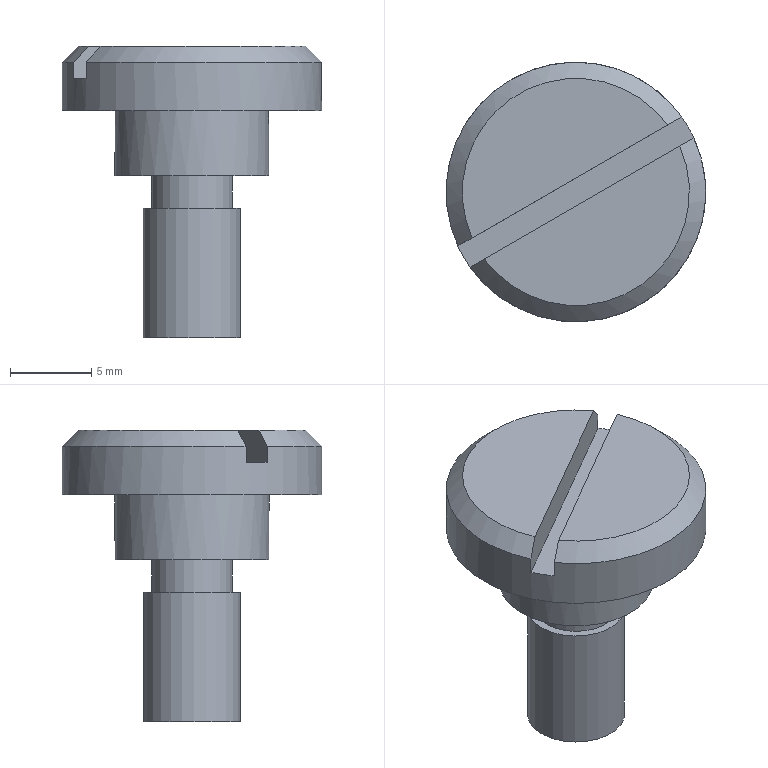Component | NX | DRILL_BUSH_SCREW | 1 solid | 15 faces | box 16 x 16 x 18 mm | volume 1283 mm3 | plane 9 | cylinder 4 | cone 2 | commonest cylinder face diameters 6 x1 5 x1 9.5 x1 16 x1
STEP:
#1=CARTESIAN_POINT('',(0.,0.,0.));
#2=DIRECTION('',(0.,0.,1.));
#3=DIRECTION('',(1.,0.,0.));
#4=AXIS2_PLACEMENT_3D('',#1,#2,#3);
#5=CARTESIAN_POINT('',(-27.652,33.976,178.));
#6=VERTEX_POINT('',#5);
#7=CARTESIAN_POINT('',(-15.598,40.935,178.));
#8=VERTEX_POINT('',#7);
#9=CARTESIAN_POINT('',(-31.151,31.956,178.));
#10=DIRECTION('',(0.866,0.5,0.));
#11=VECTOR('',#10,1.);
#12=LINE('',#9,#11);
#13=CARTESIAN_POINT('',(-22.,38.105,178.));
#14=DIRECTION('',(0.,0.,1.));
#15=DIRECTION('',(0.866,0.5,0.));
#16=AXIS2_PLACEMENT_3D('',#13,#14,#15);
#17=PLANE('',#16);
#18=CARTESIAN_POINT('',(-11.,-0.75));
#19=DIRECTION('',(1.,0.));
#20=VECTOR('',#19,1.);
#21=LINE('',#18,#20);
#22=(GEOMETRIC_REPRESENTATION_CONTEXT(2)PARAMETRIC_REPRESENTATION_CONTEXT()REPRESENTATION_CONTEXT('',''));
#23=DEFINITIONAL_REPRESENTATION('',(#21),#22);
#24=PCURVE('',#17,#23);
#25=CARTESIAN_POINT('',(-31.151,31.956,176.));
#26=DIRECTION('',(0.5,-0.866,0.));
#27=DIRECTION('',(0.,0.,-1.));
#28=AXIS2_PLACEMENT_3D('',#25,#26,#27);
#29=PLANE('',#28);
#30=CARTESIAN_POINT('',(-2.,0.));
#31=DIRECTION('',(0.,1.));
#32=VECTOR('',#31,1.);
#33=LINE('',#30,#32);
#34=(GEOMETRIC_REPRESENTATION_CONTEXT(2)PARAMETRIC_REPRESENTATION_CONTEXT()REPRESENTATION_CONTEXT('',''));
#35=DEFINITIONAL_REPRESENTATION('',(#33),#34);
#36=PCURVE('',#29,#35);
#37=SURFACE_CURVE('',#12,(#24,#36),.PCURVE_S1.);
#38=EDGE_CURVE('',#6,#8,#37,.T.);
#39=ORIENTED_EDGE('',*,*,#38,.F.);
#40=CARTESIAN_POINT('',(-22.,38.105,178.));
#41=DIRECTION('',(0.,0.,1.));
#42=DIRECTION('',(0.866,0.5,0.));
#43=AXIS2_PLACEMENT_3D('',#40,#41,#42);
#44=CIRCLE('',#43,7.);
#45=CARTESIAN_POINT('',(0.,0.));
#46=DIRECTION('',(1.,0.));
#47=AXIS2_PLACEMENT_2D('',#45,#46);
#48=CIRCLE('',#47,7.);
#49=(GEOMETRIC_REPRESENTATION_CONTEXT(2)PARAMETRIC_REPRESENTATION_CONTEXT()REPRESENTATION_CONTEXT('',''));
#50=DEFINITIONAL_REPRESENTATION('',(#48),#49);
#51=PCURVE('',#17,#50);
#52=CARTESIAN_POINT('',(-22.,38.105,177.));
#53=DIRECTION('',(0.,0.,-1.));
#54=DIRECTION('',(-0.866,-0.5,0.));
#55=AXIS2_PLACEMENT_3D('',#52,#53,#54);
#56=CONICAL_SURFACE('',#55,8.,0.7854);
#57=CARTESIAN_POINT('',(9.425,-1.));
#58=DIRECTION('',(-1.,0.));
#59=VECTOR('',#58,1.);
#60=LINE('',#57,#59);
#61=(GEOMETRIC_REPRESENTATION_CONTEXT(2)PARAMETRIC_REPRESENTATION_CONTEXT()REPRESENTATION_CONTEXT('',''));
#62=DEFINITIONAL_REPRESENTATION('',(#60),#61);
#63=PCURVE('',#56,#62);
#64=SURFACE_CURVE('',#44,(#51,#63),.PCURVE_S1.);
#65=EDGE_CURVE('',#6,#8,#64,.T.);
#66=ORIENTED_EDGE('',*,*,#65,.T.);
#67=EDGE_LOOP('',(#39,#66));
#68=FACE_BOUND('',#67,.T.);
#69=ADVANCED_FACE('',(#68),#17,.T.);
#70=CARTESIAN_POINT('',(-19.835,39.355,168.));
#71=VERTEX_POINT('',#70);
#72=CARTESIAN_POINT('',(-22.,38.105,168.));
#73=DIRECTION('',(0.,0.,1.));
#74=DIRECTION('',(0.866,0.5,0.));
#75=AXIS2_PLACEMENT_3D('',#72,#73,#74);
#76=CIRCLE('',#75,2.5);
#77=CARTESIAN_POINT('',(-22.,38.105,168.));
#78=DIRECTION('',(0.,0.,1.));
#79=DIRECTION('',(0.866,0.5,0.));
#80=AXIS2_PLACEMENT_3D('',#77,#78,#79);
#81=PLANE('',#80);
#82=CARTESIAN_POINT('',(0.,0.));
#83=DIRECTION('',(1.,-0.));
#84=AXIS2_PLACEMENT_2D('',#82,#83);
#85=CIRCLE('',#84,2.5);
#86=(GEOMETRIC_REPRESENTATION_CONTEXT(2)PARAMETRIC_REPRESENTATION_CONTEXT()REPRESENTATION_CONTEXT('',''));
#87=DEFINITIONAL_REPRESENTATION('',(#85),#86);
#88=PCURVE('',#81,#87);
#89=CARTESIAN_POINT('',(-22.,38.105,168.));
#90=DIRECTION('',(0.,0.,1.));
#91=DIRECTION('',(0.866,0.5,0.));
#92=AXIS2_PLACEMENT_3D('',#89,#90,#91);
#93=CYLINDRICAL_SURFACE('',#92,2.5);
#94=CARTESIAN_POINT('',(0.,0.));
#95=DIRECTION('',(1.,0.));
#96=VECTOR('',#95,1.);
#97=LINE('',#94,#96);
#98=(GEOMETRIC_REPRESENTATION_CONTEXT(2)PARAMETRIC_REPRESENTATION_CONTEXT()REPRESENTATION_CONTEXT('',''));
#99=DEFINITIONAL_REPRESENTATION('',(#97),#98);
#100=PCURVE('',#93,#99);
#101=SURFACE_CURVE('',#76,(#88,#100),.PCURVE_S1.);
#102=EDGE_CURVE('',#71,#71,#101,.T.);
#103=ORIENTED_EDGE('',*,*,#102,.F.);
#104=EDGE_LOOP('',(#103));
#105=FACE_BOUND('',#104,.T.);
#106=CARTESIAN_POINT('',(-19.402,39.605,168.));
#107=VERTEX_POINT('',#106);
#108=CARTESIAN_POINT('',(-22.,38.105,168.));
#109=DIRECTION('',(0.,0.,-1.));
#110=DIRECTION('',(0.866,0.5,0.));
#111=AXIS2_PLACEMENT_3D('',#108,#109,#110);
#112=CIRCLE('',#111,3.);
#113=CARTESIAN_POINT('',(3.,0.));
#114=CARTESIAN_POINT('',(3.,-5.196));
#115=CARTESIAN_POINT('',(-1.5,-2.598));
#116=CARTESIAN_POINT('',(-6.,-0.));
#117=CARTESIAN_POINT('',(-1.5,2.598));
#118=CARTESIAN_POINT('',(3.,5.196));
#119=CARTESIAN_POINT('',(3.,0.));
#120=(BOUNDED_CURVE()B_SPLINE_CURVE(2,(#113,#114,#115,#116,#117,#118,#119),.UNSPECIFIED.,.T.,.F.)B_SPLINE_CURVE_WITH_KNOTS((1,2,2,2,2,1),(-2.094,0.,2.094,4.189,6.283,8.378),.UNSPECIFIED.)CURVE()GEOMETRIC_REPRESENTATION_ITEM()RATIONAL_B_SPLINE_CURVE((1.,0.5,1.,0.5,1.,0.5,1.))REPRESENTATION_ITEM(''));
#121=(GEOMETRIC_REPRESENTATION_CONTEXT(2)PARAMETRIC_REPRESENTATION_CONTEXT()REPRESENTATION_CONTEXT('',''));
#122=DEFINITIONAL_REPRESENTATION('',(#120),#121);
#123=PCURVE('',#81,#122);
#124=CARTESIAN_POINT('',(-22.,38.105,160.));
#125=DIRECTION('',(0.,0.,1.));
#126=DIRECTION('',(0.866,0.5,0.));
#127=AXIS2_PLACEMENT_3D('',#124,#125,#126);
#128=CYLINDRICAL_SURFACE('',#127,3.);
#129=CARTESIAN_POINT('',(6.283,8.));
#130=DIRECTION('',(-1.,0.));
#131=VECTOR('',#130,1.);
#132=LINE('',#129,#131);
#133=(GEOMETRIC_REPRESENTATION_CONTEXT(2)PARAMETRIC_REPRESENTATION_CONTEXT()REPRESENTATION_CONTEXT('',''));
#134=DEFINITIONAL_REPRESENTATION('',(#132),#133);
#135=PCURVE('',#128,#134);
#136=SURFACE_CURVE('',#112,(#123,#135),.PCURVE_S1.);
#137=EDGE_CURVE('',#107,#107,#136,.T.);
#138=ORIENTED_EDGE('',*,*,#137,.F.);
#139=EDGE_LOOP('',(#138));
#140=FACE_BOUND('',#139,.T.);
#141=ADVANCED_FACE('',(#105,#140),#81,.T.);
#142=CARTESIAN_POINT('',(-19.402,39.605,160.));
#143=VERTEX_POINT('',#142);
#144=CARTESIAN_POINT('',(-22.,38.105,160.));
#145=DIRECTION('',(0.,0.,1.));
#146=DIRECTION('',(0.866,0.5,0.));
#147=AXIS2_PLACEMENT_3D('',#144,#145,#146);
#148=CIRCLE('',#147,3.);
#149=CARTESIAN_POINT('',(-22.,38.105,160.));
#150=DIRECTION('',(0.,0.,-1.));
#151=DIRECTION('',(-0.866,-0.5,0.));
#152=AXIS2_PLACEMENT_3D('',#149,#150,#151);
#153=PLANE('',#152);
#154=CARTESIAN_POINT('',(-3.,0.));
#155=CARTESIAN_POINT('',(-3.,5.196));
#156=CARTESIAN_POINT('',(1.5,2.598));
#157=CARTESIAN_POINT('',(6.,-0.));
#158=CARTESIAN_POINT('',(1.5,-2.598));
#159=CARTESIAN_POINT('',(-3.,-5.196));
#160=CARTESIAN_POINT('',(-3.,0.));
#161=(BOUNDED_CURVE()B_SPLINE_CURVE(2,(#154,#155,#156,#157,#158,#159,#160),.UNSPECIFIED.,.T.,.F.)B_SPLINE_CURVE_WITH_KNOTS((1,2,2,2,2,1),(-2.094,0.,2.094,4.189,6.283,8.378),.UNSPECIFIED.)CURVE()GEOMETRIC_REPRESENTATION_ITEM()RATIONAL_B_SPLINE_CURVE((1.,0.5,1.,0.5,1.,0.5,1.))REPRESENTATION_ITEM(''));
#162=(GEOMETRIC_REPRESENTATION_CONTEXT(2)PARAMETRIC_REPRESENTATION_CONTEXT()REPRESENTATION_CONTEXT('',''));
#163=DEFINITIONAL_REPRESENTATION('',(#161),#162);
#164=PCURVE('',#153,#163);
#165=CARTESIAN_POINT('',(0.,0.));
#166=DIRECTION('',(1.,0.));
#167=VECTOR('',#166,1.);
#168=LINE('',#165,#167);
#169=(GEOMETRIC_REPRESENTATION_CONTEXT(2)PARAMETRIC_REPRESENTATION_CONTEXT()REPRESENTATION_CONTEXT('',''));
#170=DEFINITIONAL_REPRESENTATION('',(#168),#169);
#171=PCURVE('',#128,#170);
#172=SURFACE_CURVE('',#148,(#164,#171),.PCURVE_S1.);
#173=EDGE_CURVE('',#143,#143,#172,.T.);
#174=ORIENTED_EDGE('',*,*,#173,.F.);
#175=EDGE_LOOP('',(#174));
#176=FACE_BOUND('',#175,.T.);
#177=ADVANCED_FACE('',(#176),#153,.T.);
#178=ORIENTED_EDGE('',*,*,#137,.T.);
#179=CARTESIAN_POINT('',(-19.402,39.605,160.));
#180=CARTESIAN_POINT('',(-19.402,39.605,168.));
#181=B_SPLINE_CURVE_WITH_KNOTS('',1,(#179,#180),.UNSPECIFIED.,.F.,.F.,(2,2),(0.,8.),.PIECEWISE_BEZIER_KNOTS.);
#182=CARTESIAN_POINT('',(0.,0.));
#183=DIRECTION('',(0.,1.));
#184=VECTOR('',#183,1.);
#185=LINE('',#182,#184);
#186=(GEOMETRIC_REPRESENTATION_CONTEXT(2)PARAMETRIC_REPRESENTATION_CONTEXT()REPRESENTATION_CONTEXT('',''));
#187=DEFINITIONAL_REPRESENTATION('',(#185),#186);
#188=PCURVE('',#128,#187);
#189=CARTESIAN_POINT('',(6.283,0.));
#190=DIRECTION('',(0.,1.));
#191=VECTOR('',#190,1.);
#192=LINE('',#189,#191);
#193=(GEOMETRIC_REPRESENTATION_CONTEXT(2)PARAMETRIC_REPRESENTATION_CONTEXT()REPRESENTATION_CONTEXT('',''));
#194=DEFINITIONAL_REPRESENTATION('',(#192),#193);
#195=PCURVE('',#128,#194);
#196=SEAM_CURVE('',#181,(#188,#195),.PCURVE_S1.);
#197=EDGE_CURVE('',#143,#107,#196,.T.);
#198=ORIENTED_EDGE('',*,*,#197,.F.);
#199=ORIENTED_EDGE('',*,*,#173,.T.);
#200=ORIENTED_EDGE('',*,*,#197,.T.);
#201=EDGE_LOOP('',(#178,#198,#199,#200));
#202=FACE_BOUND('',#201,.T.);
#203=ADVANCED_FACE('',(#202),#128,.T.);
#204=CARTESIAN_POINT('',(-19.835,39.355,170.));
#205=VERTEX_POINT('',#204);
#206=CARTESIAN_POINT('',(-24.165,36.855,170.));
#207=VERTEX_POINT('',#206);
#208=CARTESIAN_POINT('',(-22.,38.105,170.));
#209=DIRECTION('',(0.,0.,1.));
#210=DIRECTION('',(-0.866,-0.5,0.));
#211=AXIS2_PLACEMENT_3D('',#208,#209,#210);
#212=CIRCLE('',#211,2.5);
#213=CARTESIAN_POINT('',(-3.142,2.));
#214=DIRECTION('',(1.,0.));
#215=VECTOR('',#214,1.);
#216=LINE('',#213,#215);
#217=(GEOMETRIC_REPRESENTATION_CONTEXT(2)PARAMETRIC_REPRESENTATION_CONTEXT()REPRESENTATION_CONTEXT('',''));
#218=DEFINITIONAL_REPRESENTATION('',(#216),#217);
#219=PCURVE('',#93,#218);
#220=CARTESIAN_POINT('',(-22.,38.105,170.));
#221=DIRECTION('',(0.,0.,-1.));
#222=DIRECTION('',(-0.866,-0.5,0.));
#223=AXIS2_PLACEMENT_3D('',#220,#221,#222);
#224=PLANE('',#223);
#225=CARTESIAN_POINT('',(2.5,0.));
#226=CARTESIAN_POINT('',(2.5,-4.33));
#227=CARTESIAN_POINT('',(-1.25,-2.165));
#228=CARTESIAN_POINT('',(-5.,-0.));
#229=CARTESIAN_POINT('',(-1.25,2.165));
#230=CARTESIAN_POINT('',(2.5,4.33));
#231=CARTESIAN_POINT('',(2.5,0.));
#232=(BOUNDED_CURVE()B_SPLINE_CURVE(2,(#225,#226,#227,#228,#229,#230,#231),.UNSPECIFIED.,.T.,.F.)B_SPLINE_CURVE_WITH_KNOTS((1,2,2,2,2,1),(-2.094,0.,2.094,4.189,6.283,8.378),.UNSPECIFIED.)CURVE()GEOMETRIC_REPRESENTATION_ITEM()RATIONAL_B_SPLINE_CURVE((1.,0.5,1.,0.5,1.,0.5,1.))REPRESENTATION_ITEM(''));
#233=(GEOMETRIC_REPRESENTATION_CONTEXT(2)PARAMETRIC_REPRESENTATION_CONTEXT()REPRESENTATION_CONTEXT('',''));
#234=DEFINITIONAL_REPRESENTATION('',(#232),#233);
#235=PCURVE('',#224,#234);
#236=SURFACE_CURVE('',#212,(#219,#235),.PCURVE_S1.);
#237=EDGE_CURVE('',#205,#207,#236,.T.);
#238=ORIENTED_EDGE('',*,*,#237,.F.);
#239=CARTESIAN_POINT('',(-19.835,39.355,168.));
#240=CARTESIAN_POINT('',(-19.835,39.355,170.));
#241=B_SPLINE_CURVE_WITH_KNOTS('',1,(#239,#240),.UNSPECIFIED.,.F.,.F.,(2,2),(0.,2.),.PIECEWISE_BEZIER_KNOTS.);
#242=CARTESIAN_POINT('',(0.,0.));
#243=DIRECTION('',(0.,1.));
#244=VECTOR('',#243,1.);
#245=LINE('',#242,#244);
#246=(GEOMETRIC_REPRESENTATION_CONTEXT(2)PARAMETRIC_REPRESENTATION_CONTEXT()REPRESENTATION_CONTEXT('',''));
#247=DEFINITIONAL_REPRESENTATION('',(#245),#246);
#248=PCURVE('',#93,#247);
#249=CARTESIAN_POINT('',(6.283,0.));
#250=DIRECTION('',(0.,1.));
#251=VECTOR('',#250,1.);
#252=LINE('',#249,#251);
#253=(GEOMETRIC_REPRESENTATION_CONTEXT(2)PARAMETRIC_REPRESENTATION_CONTEXT()REPRESENTATION_CONTEXT('',''));
#254=DEFINITIONAL_REPRESENTATION('',(#252),#253);
#255=PCURVE('',#93,#254);
#256=SEAM_CURVE('',#241,(#248,#255),.PCURVE_S1.);
#257=EDGE_CURVE('',#71,#205,#256,.T.);
#258=ORIENTED_EDGE('',*,*,#257,.F.);
#259=ORIENTED_EDGE('',*,*,#102,.T.);
#260=ORIENTED_EDGE('',*,*,#257,.T.);
#261=CARTESIAN_POINT('',(-22.,38.105,170.));
#262=DIRECTION('',(0.,0.,1.));
#263=DIRECTION('',(-0.866,-0.5,0.));
#264=AXIS2_PLACEMENT_3D('',#261,#262,#263);
#265=CIRCLE('',#264,2.5);
#266=CARTESIAN_POINT('',(3.142,2.));
#267=DIRECTION('',(1.,0.));
#268=VECTOR('',#267,1.);
#269=LINE('',#266,#268);
#270=(GEOMETRIC_REPRESENTATION_CONTEXT(2)PARAMETRIC_REPRESENTATION_CONTEXT()REPRESENTATION_CONTEXT('',''));
#271=DEFINITIONAL_REPRESENTATION('',(#269),#270);
#272=PCURVE('',#93,#271);
#273=CARTESIAN_POINT('',(2.5,0.));
#274=CARTESIAN_POINT('',(2.5,-4.33));
#275=CARTESIAN_POINT('',(-1.25,-2.165));
#276=CARTESIAN_POINT('',(-5.,-0.));
#277=CARTESIAN_POINT('',(-1.25,2.165));
#278=CARTESIAN_POINT('',(2.5,4.33));
#279=CARTESIAN_POINT('',(2.5,0.));
#280=(BOUNDED_CURVE()B_SPLINE_CURVE(2,(#273,#274,#275,#276,#277,#278,#279),.UNSPECIFIED.,.T.,.F.)B_SPLINE_CURVE_WITH_KNOTS((1,2,2,2,2,1),(-2.094,0.,2.094,4.189,6.283,8.378),.UNSPECIFIED.)CURVE()GEOMETRIC_REPRESENTATION_ITEM()RATIONAL_B_SPLINE_CURVE((1.,0.5,1.,0.5,1.,0.5,1.))REPRESENTATION_ITEM(''));
#281=(GEOMETRIC_REPRESENTATION_CONTEXT(2)PARAMETRIC_REPRESENTATION_CONTEXT()REPRESENTATION_CONTEXT('',''));
#282=DEFINITIONAL_REPRESENTATION('',(#280),#281);
#283=PCURVE('',#224,#282);
#284=SURFACE_CURVE('',#265,(#272,#283),.PCURVE_S1.);
#285=EDGE_CURVE('',#207,#205,#284,.T.);
#286=ORIENTED_EDGE('',*,*,#285,.F.);
#287=EDGE_LOOP('',(#238,#258,#259,#260,#286));
#288=FACE_BOUND('',#287,.T.);
#289=ADVANCED_FACE('',(#288),#93,.T.);
#290=ORIENTED_EDGE('',*,*,#285,.T.);
#291=ORIENTED_EDGE('',*,*,#237,.T.);
#292=EDGE_LOOP('',(#290,#291));
#293=FACE_BOUND('',#292,.T.);
#294=CARTESIAN_POINT('',(-17.886,40.48,170.));
#295=VERTEX_POINT('',#294);
#296=CARTESIAN_POINT('',(-22.,38.105,170.));
#297=DIRECTION('',(0.,0.,1.));
#298=DIRECTION('',(0.866,0.5,0.));
#299=AXIS2_PLACEMENT_3D('',#296,#297,#298);
#300=CIRCLE('',#299,4.75);
#301=CARTESIAN_POINT('',(-4.75,0.));
#302=CARTESIAN_POINT('',(-4.75,8.227));
#303=CARTESIAN_POINT('',(2.375,4.114));
#304=CARTESIAN_POINT('',(9.5,0.));
#305=CARTESIAN_POINT('',(2.375,-4.114));
#306=CARTESIAN_POINT('',(-4.75,-8.227));
#307=CARTESIAN_POINT('',(-4.75,0.));
#308=(BOUNDED_CURVE()B_SPLINE_CURVE(2,(#301,#302,#303,#304,#305,#306,#307),.UNSPECIFIED.,.T.,.F.)B_SPLINE_CURVE_WITH_KNOTS((1,2,2,2,2,1),(-2.094,0.,2.094,4.189,6.283,8.378),.UNSPECIFIED.)CURVE()GEOMETRIC_REPRESENTATION_ITEM()RATIONAL_B_SPLINE_CURVE((1.,0.5,1.,0.5,1.,0.5,1.))REPRESENTATION_ITEM(''));
#309=(GEOMETRIC_REPRESENTATION_CONTEXT(2)PARAMETRIC_REPRESENTATION_CONTEXT()REPRESENTATION_CONTEXT('',''));
#310=DEFINITIONAL_REPRESENTATION('',(#308),#309);
#311=PCURVE('',#224,#310);
#312=CARTESIAN_POINT('',(-22.,38.105,170.));
#313=DIRECTION('',(0.,0.,1.));
#314=DIRECTION('',(0.866,0.5,0.));
#315=AXIS2_PLACEMENT_3D('',#312,#313,#314);
#316=CYLINDRICAL_SURFACE('',#315,4.75);
#317=CARTESIAN_POINT('',(0.,0.));
#318=DIRECTION('',(1.,0.));
#319=VECTOR('',#318,1.);
#320=LINE('',#317,#319);
#321=(GEOMETRIC_REPRESENTATION_CONTEXT(2)PARAMETRIC_REPRESENTATION_CONTEXT()REPRESENTATION_CONTEXT('',''));
#322=DEFINITIONAL_REPRESENTATION('',(#320),#321);
#323=PCURVE('',#316,#322);
#324=SURFACE_CURVE('',#300,(#311,#323),.PCURVE_S1.);
#325=EDGE_CURVE('',#295,#295,#324,.T.);
#326=ORIENTED_EDGE('',*,*,#325,.F.);
#327=EDGE_LOOP('',(#326));
#328=FACE_BOUND('',#327,.T.);
#329=ADVANCED_FACE('',(#293,#328),#224,.T.);
#330=CARTESIAN_POINT('',(-17.886,40.48,174.));
#331=VERTEX_POINT('',#330);
#332=CARTESIAN_POINT('',(-26.114,35.73,174.));
#333=VERTEX_POINT('',#332);
#334=CARTESIAN_POINT('',(-22.,38.105,174.));
#335=DIRECTION('',(0.,0.,1.));
#336=DIRECTION('',(-0.866,-0.5,0.));
#337=AXIS2_PLACEMENT_3D('',#334,#335,#336);
#338=CIRCLE('',#337,4.75);
#339=CARTESIAN_POINT('',(-3.142,4.));
#340=DIRECTION('',(1.,0.));
#341=VECTOR('',#340,1.);
#342=LINE('',#339,#341);
#343=(GEOMETRIC_REPRESENTATION_CONTEXT(2)PARAMETRIC_REPRESENTATION_CONTEXT()REPRESENTATION_CONTEXT('',''));
#344=DEFINITIONAL_REPRESENTATION('',(#342),#343);
#345=PCURVE('',#316,#344);
#346=CARTESIAN_POINT('',(-22.,38.105,174.));
#347=DIRECTION('',(0.,0.,-1.));
#348=DIRECTION('',(-0.866,-0.5,0.));
#349=AXIS2_PLACEMENT_3D('',#346,#347,#348);
#350=PLANE('',#349);
#351=CARTESIAN_POINT('',(4.75,0.));
#352=CARTESIAN_POINT('',(4.75,-8.227));
#353=CARTESIAN_POINT('',(-2.375,-4.114));
#354=CARTESIAN_POINT('',(-9.5,-0.));
#355=CARTESIAN_POINT('',(-2.375,4.114));
#356=CARTESIAN_POINT('',(4.75,8.227));
#357=CARTESIAN_POINT('',(4.75,0.));
#358=(BOUNDED_CURVE()B_SPLINE_CURVE(2,(#351,#352,#353,#354,#355,#356,#357),.UNSPECIFIED.,.T.,.F.)B_SPLINE_CURVE_WITH_KNOTS((1,2,2,2,2,1),(-2.094,0.,2.094,4.189,6.283,8.378),.UNSPECIFIED.)CURVE()GEOMETRIC_REPRESENTATION_ITEM()RATIONAL_B_SPLINE_CURVE((1.,0.5,1.,0.5,1.,0.5,1.))REPRESENTATION_ITEM(''));
#359=(GEOMETRIC_REPRESENTATION_CONTEXT(2)PARAMETRIC_REPRESENTATION_CONTEXT()REPRESENTATION_CONTEXT('',''));
#360=DEFINITIONAL_REPRESENTATION('',(#358),#359);
#361=PCURVE('',#350,#360);
#362=SURFACE_CURVE('',#338,(#345,#361),.PCURVE_S1.);
#363=EDGE_CURVE('',#331,#333,#362,.T.);
#364=ORIENTED_EDGE('',*,*,#363,.F.);
#365=CARTESIAN_POINT('',(-17.886,40.48,170.));
#366=CARTESIAN_POINT('',(-17.886,40.48,174.));
#367=B_SPLINE_CURVE_WITH_KNOTS('',1,(#365,#366),.UNSPECIFIED.,.F.,.F.,(2,2),(0.,4.),.PIECEWISE_BEZIER_KNOTS.);
#368=CARTESIAN_POINT('',(0.,0.));
#369=DIRECTION('',(0.,1.));
#370=VECTOR('',#369,1.);
#371=LINE('',#368,#370);
#372=(GEOMETRIC_REPRESENTATION_CONTEXT(2)PARAMETRIC_REPRESENTATION_CONTEXT()REPRESENTATION_CONTEXT('',''));
#373=DEFINITIONAL_REPRESENTATION('',(#371),#372);
#374=PCURVE('',#316,#373);
#375=CARTESIAN_POINT('',(6.283,0.));
#376=DIRECTION('',(0.,1.));
#377=VECTOR('',#376,1.);
#378=LINE('',#375,#377);
#379=(GEOMETRIC_REPRESENTATION_CONTEXT(2)PARAMETRIC_REPRESENTATION_CONTEXT()REPRESENTATION_CONTEXT('',''));
#380=DEFINITIONAL_REPRESENTATION('',(#378),#379);
#381=PCURVE('',#316,#380);
#382=SEAM_CURVE('',#367,(#374,#381),.PCURVE_S1.);
#383=EDGE_CURVE('',#295,#331,#382,.T.);
#384=ORIENTED_EDGE('',*,*,#383,.F.);
#385=ORIENTED_EDGE('',*,*,#325,.T.);
#386=ORIENTED_EDGE('',*,*,#383,.T.);
#387=CARTESIAN_POINT('',(-22.,38.105,174.));
#388=DIRECTION('',(0.,0.,1.));
#389=DIRECTION('',(-0.866,-0.5,0.));
#390=AXIS2_PLACEMENT_3D('',#387,#388,#389);
#391=CIRCLE('',#390,4.75);
#392=CARTESIAN_POINT('',(3.142,4.));
#393=DIRECTION('',(1.,0.));
#394=VECTOR('',#393,1.);
#395=LINE('',#392,#394);
#396=(GEOMETRIC_REPRESENTATION_CONTEXT(2)PARAMETRIC_REPRESENTATION_CONTEXT()REPRESENTATION_CONTEXT('',''));
#397=DEFINITIONAL_REPRESENTATION('',(#395),#396);
#398=PCURVE('',#316,#397);
#399=CARTESIAN_POINT('',(4.75,0.));
#400=CARTESIAN_POINT('',(4.75,-8.227));
#401=CARTESIAN_POINT('',(-2.375,-4.114));
#402=CARTESIAN_POINT('',(-9.5,-0.));
#403=CARTESIAN_POINT('',(-2.375,4.114));
#404=CARTESIAN_POINT('',(4.75,8.227));
#405=CARTESIAN_POINT('',(4.75,0.));
#406=(BOUNDED_CURVE()B_SPLINE_CURVE(2,(#399,#400,#401,#402,#403,#404,#405),.UNSPECIFIED.,.T.,.F.)B_SPLINE_CURVE_WITH_KNOTS((1,2,2,2,2,1),(-2.094,0.,2.094,4.189,6.283,8.378),.UNSPECIFIED.)CURVE()GEOMETRIC_REPRESENTATION_ITEM()RATIONAL_B_SPLINE_CURVE((1.,0.5,1.,0.5,1.,0.5,1.))REPRESENTATION_ITEM(''));
#407=(GEOMETRIC_REPRESENTATION_CONTEXT(2)PARAMETRIC_REPRESENTATION_CONTEXT()REPRESENTATION_CONTEXT('',''));
#408=DEFINITIONAL_REPRESENTATION('',(#406),#407);
#409=PCURVE('',#350,#408);
#410=SURFACE_CURVE('',#391,(#398,#409),.PCURVE_S1.);
#411=EDGE_CURVE('',#333,#331,#410,.T.);
#412=ORIENTED_EDGE('',*,*,#411,.F.);
#413=EDGE_LOOP('',(#364,#384,#385,#386,#412));
#414=FACE_BOUND('',#413,.T.);
#415=ADVANCED_FACE('',(#414),#316,.T.);
#416=CARTESIAN_POINT('',(-16.348,42.234,178.));
#417=VERTEX_POINT('',#416);
#418=CARTESIAN_POINT('',(-28.402,35.275,178.));
#419=VERTEX_POINT('',#418);
#420=CARTESIAN_POINT('',(-12.849,44.255,178.));
#421=DIRECTION('',(-0.866,-0.5,0.));
#422=VECTOR('',#421,1.);
#423=LINE('',#420,#422);
#424=CARTESIAN_POINT('',(-22.,38.105,178.));
#425=DIRECTION('',(0.,0.,1.));
#426=DIRECTION('',(0.866,0.5,0.));
#427=AXIS2_PLACEMENT_3D('',#424,#425,#426);
#428=PLANE('',#427);
#429=CARTESIAN_POINT('',(11.,0.75));
#430=DIRECTION('',(-1.,0.));
#431=VECTOR('',#430,1.);
#432=LINE('',#429,#431);
#433=(GEOMETRIC_REPRESENTATION_CONTEXT(2)PARAMETRIC_REPRESENTATION_CONTEXT()REPRESENTATION_CONTEXT('',''));
#434=DEFINITIONAL_REPRESENTATION('',(#432),#433);
#435=PCURVE('',#428,#434);
#436=CARTESIAN_POINT('',(-12.849,44.255,176.));
#437=DIRECTION('',(-0.5,0.866,0.));
#438=DIRECTION('',(0.,0.,1.));
#439=AXIS2_PLACEMENT_3D('',#436,#437,#438);
#440=PLANE('',#439);
#441=CARTESIAN_POINT('',(2.,0.));
#442=DIRECTION('',(0.,-1.));
#443=VECTOR('',#442,1.);
#444=LINE('',#441,#443);
#445=(GEOMETRIC_REPRESENTATION_CONTEXT(2)PARAMETRIC_REPRESENTATION_CONTEXT()REPRESENTATION_CONTEXT('',''));
#446=DEFINITIONAL_REPRESENTATION('',(#444),#445);
#447=PCURVE('',#440,#446);
#448=SURFACE_CURVE('',#423,(#435,#447),.PCURVE_S1.);
#449=EDGE_CURVE('',#417,#419,#448,.T.);
#450=ORIENTED_EDGE('',*,*,#449,.F.);
#451=CARTESIAN_POINT('',(-22.,38.105,178.));
#452=DIRECTION('',(0.,0.,1.));
#453=DIRECTION('',(0.866,0.5,0.));
#454=AXIS2_PLACEMENT_3D('',#451,#452,#453);
#455=CIRCLE('',#454,7.);
#456=CARTESIAN_POINT('',(0.,0.));
#457=DIRECTION('',(1.,0.));
#458=AXIS2_PLACEMENT_2D('',#456,#457);
#459=CIRCLE('',#458,7.);
#460=(GEOMETRIC_REPRESENTATION_CONTEXT(2)PARAMETRIC_REPRESENTATION_CONTEXT()REPRESENTATION_CONTEXT('',''));
#461=DEFINITIONAL_REPRESENTATION('',(#459),#460);
#462=PCURVE('',#428,#461);
#463=CARTESIAN_POINT('',(-22.,38.105,177.));
#464=DIRECTION('',(0.,0.,-1.));
#465=DIRECTION('',(-0.866,-0.5,0.));
#466=AXIS2_PLACEMENT_3D('',#463,#464,#465);
#467=CONICAL_SURFACE('',#466,8.,0.7854);
#468=CARTESIAN_POINT('',(3.142,-1.));
#469=DIRECTION('',(-1.,0.));
#470=VECTOR('',#469,1.);
#471=LINE('',#468,#470);
#472=(GEOMETRIC_REPRESENTATION_CONTEXT(2)PARAMETRIC_REPRESENTATION_CONTEXT()REPRESENTATION_CONTEXT('',''));
#473=DEFINITIONAL_REPRESENTATION('',(#471),#472);
#474=PCURVE('',#467,#473);
#475=SURFACE_CURVE('',#455,(#462,#474),.PCURVE_S1.);
#476=EDGE_CURVE('',#417,#419,#475,.T.);
#477=ORIENTED_EDGE('',*,*,#476,.T.);
#478=EDGE_LOOP('',(#450,#477));
#479=FACE_BOUND('',#478,.T.);
#480=ADVANCED_FACE('',(#479),#428,.T.);
#481=ORIENTED_EDGE('',*,*,#411,.T.);
#482=ORIENTED_EDGE('',*,*,#363,.T.);
#483=EDGE_LOOP('',(#481,#482));
#484=FACE_BOUND('',#483,.T.);
#485=CARTESIAN_POINT('',(-15.072,42.105,174.));
#486=VERTEX_POINT('',#485);
#487=CARTESIAN_POINT('',(-22.,38.105,174.));
#488=DIRECTION('',(0.,0.,1.));
#489=DIRECTION('',(0.866,0.5,0.));
#490=AXIS2_PLACEMENT_3D('',#487,#488,#489);
#491=CIRCLE('',#490,8.);
#492=CARTESIAN_POINT('',(-8.,0.));
#493=CARTESIAN_POINT('',(-8.,13.856));
#494=CARTESIAN_POINT('',(4.,6.928));
#495=CARTESIAN_POINT('',(16.,0.));
#496=CARTESIAN_POINT('',(4.,-6.928));
#497=CARTESIAN_POINT('',(-8.,-13.856));
#498=CARTESIAN_POINT('',(-8.,0.));
#499=(BOUNDED_CURVE()B_SPLINE_CURVE(2,(#492,#493,#494,#495,#496,#497,#498),.UNSPECIFIED.,.T.,.F.)B_SPLINE_CURVE_WITH_KNOTS((1,2,2,2,2,1),(-2.094,0.,2.094,4.189,6.283,8.378),.UNSPECIFIED.)CURVE()GEOMETRIC_REPRESENTATION_ITEM()RATIONAL_B_SPLINE_CURVE((1.,0.5,1.,0.5,1.,0.5,1.))REPRESENTATION_ITEM(''));
#500=(GEOMETRIC_REPRESENTATION_CONTEXT(2)PARAMETRIC_REPRESENTATION_CONTEXT()REPRESENTATION_CONTEXT('',''));
#501=DEFINITIONAL_REPRESENTATION('',(#499),#500);
#502=PCURVE('',#350,#501);
#503=CARTESIAN_POINT('',(-22.,38.105,174.));
#504=DIRECTION('',(0.,0.,1.));
#505=DIRECTION('',(0.866,0.5,0.));
#506=AXIS2_PLACEMENT_3D('',#503,#504,#505);
#507=CYLINDRICAL_SURFACE('',#506,8.);
#508=CARTESIAN_POINT('',(0.,0.));
#509=DIRECTION('',(1.,0.));
#510=VECTOR('',#509,1.);
#511=LINE('',#508,#510);
#512=(GEOMETRIC_REPRESENTATION_CONTEXT(2)PARAMETRIC_REPRESENTATION_CONTEXT()REPRESENTATION_CONTEXT('',''));
#513=DEFINITIONAL_REPRESENTATION('',(#511),#512);
#514=PCURVE('',#507,#513);
#515=SURFACE_CURVE('',#491,(#502,#514),.PCURVE_S1.);
#516=EDGE_CURVE('',#486,#486,#515,.T.);
#517=ORIENTED_EDGE('',*,*,#516,.F.);
#518=EDGE_LOOP('',(#517));
#519=FACE_BOUND('',#518,.T.);
#520=ADVANCED_FACE('',(#484,#519),#350,.T.);
#521=CARTESIAN_POINT('',(-14.727,41.438,177.));
#522=VERTEX_POINT('',#521);
#523=CARTESIAN_POINT('',(-14.727,41.438,176.));
#524=VERTEX_POINT('',#523);
#525=CARTESIAN_POINT('',(-14.727,41.438,174.));
#526=DIRECTION('',(0.,0.,-1.));
#527=VECTOR('',#526,1.);
#528=LINE('',#525,#527);
#529=CARTESIAN_POINT('',(6.189,0.));
#530=DIRECTION('',(0.,-1.));
#531=VECTOR('',#530,1.);
#532=LINE('',#529,#531);
#533=(GEOMETRIC_REPRESENTATION_CONTEXT(2)PARAMETRIC_REPRESENTATION_CONTEXT()REPRESENTATION_CONTEXT('',''));
#534=DEFINITIONAL_REPRESENTATION('',(#532),#533);
#535=PCURVE('',#507,#534);
#536=CARTESIAN_POINT('',(2.,18.965));
#537=DIRECTION('',(1.,0.));
#538=VECTOR('',#537,1.);
#539=LINE('',#536,#538);
#540=(GEOMETRIC_REPRESENTATION_CONTEXT(2)PARAMETRIC_REPRESENTATION_CONTEXT()REPRESENTATION_CONTEXT('',''));
#541=DEFINITIONAL_REPRESENTATION('',(#539),#540);
#542=PCURVE('',#29,#541);
#543=SURFACE_CURVE('',#528,(#535,#542),.PCURVE_S1.);
#544=EDGE_CURVE('',#522,#524,#543,.T.);
#545=ORIENTED_EDGE('',*,*,#544,.F.);
#546=CARTESIAN_POINT('',(-28.523,33.473,177.));
#547=VERTEX_POINT('',#546);
#548=CARTESIAN_POINT('',(-22.,38.105,177.));
#549=DIRECTION('',(0.,0.,-1.));
#550=DIRECTION('',(0.866,0.5,0.));
#551=AXIS2_PLACEMENT_3D('',#548,#549,#550);
#552=CIRCLE('',#551,8.);
#553=CARTESIAN_POINT('',(6.283,3.));
#554=DIRECTION('',(-1.,0.));
#555=VECTOR('',#554,1.);
#556=LINE('',#553,#555);
#557=(GEOMETRIC_REPRESENTATION_CONTEXT(2)PARAMETRIC_REPRESENTATION_CONTEXT()REPRESENTATION_CONTEXT('',''));
#558=DEFINITIONAL_REPRESENTATION('',(#556),#557);
#559=PCURVE('',#507,#558);
#560=CARTESIAN_POINT('',(3.142,0.));
#561=DIRECTION('',(1.,-0.));
#562=VECTOR('',#561,1.);
#563=LINE('',#560,#562);
#564=(GEOMETRIC_REPRESENTATION_CONTEXT(2)PARAMETRIC_REPRESENTATION_CONTEXT()REPRESENTATION_CONTEXT('',''));
#565=DEFINITIONAL_REPRESENTATION('',(#563),#564);
#566=PCURVE('',#56,#565);
#567=SURFACE_CURVE('',#552,(#559,#566),.PCURVE_S1.);
#568=EDGE_CURVE('',#522,#547,#567,.T.);
#569=ORIENTED_EDGE('',*,*,#568,.T.);
#570=CARTESIAN_POINT('',(-28.523,33.473,176.));
#571=VERTEX_POINT('',#570);
#572=CARTESIAN_POINT('',(-28.523,33.473,174.));
#573=DIRECTION('',(0.,0.,1.));
#574=VECTOR('',#573,1.);
#575=LINE('',#572,#574);
#576=CARTESIAN_POINT('',(3.235,0.));
#577=DIRECTION('',(0.,1.));
#578=VECTOR('',#577,1.);
#579=LINE('',#576,#578);
#580=(GEOMETRIC_REPRESENTATION_CONTEXT(2)PARAMETRIC_REPRESENTATION_CONTEXT()REPRESENTATION_CONTEXT('',''));
#581=DEFINITIONAL_REPRESENTATION('',(#579),#580);
#582=PCURVE('',#507,#581);
#583=CARTESIAN_POINT('',(2.,3.035));
#584=DIRECTION('',(-1.,0.));
#585=VECTOR('',#584,1.);
#586=LINE('',#583,#585);
#587=(GEOMETRIC_REPRESENTATION_CONTEXT(2)PARAMETRIC_REPRESENTATION_CONTEXT()REPRESENTATION_CONTEXT('',''));
#588=DEFINITIONAL_REPRESENTATION('',(#586),#587);
#589=PCURVE('',#29,#588);
#590=SURFACE_CURVE('',#575,(#582,#589),.PCURVE_S1.);
#591=EDGE_CURVE('',#571,#547,#590,.T.);
#592=ORIENTED_EDGE('',*,*,#591,.F.);
#593=CARTESIAN_POINT('',(-29.273,34.772,176.));
#594=VERTEX_POINT('',#593);
#595=CARTESIAN_POINT('',(-22.,38.105,176.));
#596=DIRECTION('',(0.,0.,-1.));
#597=DIRECTION('',(0.866,0.5,0.));
#598=AXIS2_PLACEMENT_3D('',#595,#596,#597);
#599=CIRCLE('',#598,8.);
#600=CARTESIAN_POINT('',(6.283,2.));
#601=DIRECTION('',(-1.,0.));
#602=VECTOR('',#601,1.);
#603=LINE('',#600,#602);
#604=(GEOMETRIC_REPRESENTATION_CONTEXT(2)PARAMETRIC_REPRESENTATION_CONTEXT()REPRESENTATION_CONTEXT('',''));
#605=DEFINITIONAL_REPRESENTATION('',(#603),#604);
#606=PCURVE('',#507,#605);
#607=CARTESIAN_POINT('',(-22.,38.105,176.));
#608=DIRECTION('',(0.,0.,1.));
#609=DIRECTION('',(0.866,0.5,0.));
#610=AXIS2_PLACEMENT_3D('',#607,#608,#609);
#611=PLANE('',#610);
#612=CARTESIAN_POINT('',(8.,0.));
#613=CARTESIAN_POINT('',(8.,-13.856));
#614=CARTESIAN_POINT('',(-4.,-6.928));
#615=CARTESIAN_POINT('',(-16.,-0.));
#616=CARTESIAN_POINT('',(-4.,6.928));
#617=CARTESIAN_POINT('',(8.,13.856));
#618=CARTESIAN_POINT('',(8.,0.));
#619=(BOUNDED_CURVE()B_SPLINE_CURVE(2,(#612,#613,#614,#615,#616,#617,#618),.UNSPECIFIED.,.T.,.F.)B_SPLINE_CURVE_WITH_KNOTS((1,2,2,2,2,1),(-2.094,0.,2.094,4.189,6.283,8.378),.UNSPECIFIED.)CURVE()GEOMETRIC_REPRESENTATION_ITEM()RATIONAL_B_SPLINE_CURVE((1.,0.5,1.,0.5,1.,0.5,1.))REPRESENTATION_ITEM(''));
#620=(GEOMETRIC_REPRESENTATION_CONTEXT(2)PARAMETRIC_REPRESENTATION_CONTEXT()REPRESENTATION_CONTEXT('',''));
#621=DEFINITIONAL_REPRESENTATION('',(#619),#620);
#622=PCURVE('',#611,#621);
#623=SURFACE_CURVE('',#599,(#606,#622),.PCURVE_S1.);
#624=EDGE_CURVE('',#571,#594,#623,.T.);
#625=ORIENTED_EDGE('',*,*,#624,.T.);
#626=CARTESIAN_POINT('',(-29.273,34.772,177.));
#627=VERTEX_POINT('',#626);
#628=CARTESIAN_POINT('',(-29.273,34.772,174.));
#629=DIRECTION('',(0.,0.,-1.));
#630=VECTOR('',#629,1.);
#631=LINE('',#628,#630);
#632=CARTESIAN_POINT('',(3.048,0.));
#633=DIRECTION('',(0.,-1.));
#634=VECTOR('',#633,1.);
#635=LINE('',#632,#634);
#636=(GEOMETRIC_REPRESENTATION_CONTEXT(2)PARAMETRIC_REPRESENTATION_CONTEXT()REPRESENTATION_CONTEXT('',''));
#637=DEFINITIONAL_REPRESENTATION('',(#635),#636);
#638=PCURVE('',#507,#637);
#639=CARTESIAN_POINT('',(-2.,-18.965));
#640=DIRECTION('',(-1.,0.));
#641=VECTOR('',#640,1.);
#642=LINE('',#639,#641);
#643=(GEOMETRIC_REPRESENTATION_CONTEXT(2)PARAMETRIC_REPRESENTATION_CONTEXT()REPRESENTATION_CONTEXT('',''));
#644=DEFINITIONAL_REPRESENTATION('',(#642),#643);
#645=PCURVE('',#440,#644);
#646=SURFACE_CURVE('',#631,(#638,#645),.PCURVE_S1.);
#647=EDGE_CURVE('',#627,#594,#646,.T.);
#648=ORIENTED_EDGE('',*,*,#647,.F.);
#649=CARTESIAN_POINT('',(-15.477,42.737,177.));
#650=VERTEX_POINT('',#649);
#651=CARTESIAN_POINT('',(-22.,38.105,177.));
#652=DIRECTION('',(0.,0.,-1.));
#653=DIRECTION('',(0.866,0.5,0.));
#654=AXIS2_PLACEMENT_3D('',#651,#652,#653);
#655=CIRCLE('',#654,8.);
#656=CARTESIAN_POINT('',(6.283,3.));
#657=DIRECTION('',(-1.,0.));
#658=VECTOR('',#657,1.);
#659=LINE('',#656,#658);
#660=(GEOMETRIC_REPRESENTATION_CONTEXT(2)PARAMETRIC_REPRESENTATION_CONTEXT()REPRESENTATION_CONTEXT('',''));
#661=DEFINITIONAL_REPRESENTATION('',(#659),#660);
#662=PCURVE('',#507,#661);
#663=CARTESIAN_POINT('',(-3.142,-0.));
#664=DIRECTION('',(1.,0.));
#665=VECTOR('',#664,1.);
#666=LINE('',#663,#665);
#667=(GEOMETRIC_REPRESENTATION_CONTEXT(2)PARAMETRIC_REPRESENTATION_CONTEXT()REPRESENTATION_CONTEXT('',''));
#668=DEFINITIONAL_REPRESENTATION('',(#666),#667);
#669=PCURVE('',#467,#668);
#670=SURFACE_CURVE('',#655,(#662,#669),.PCURVE_S1.);
#671=EDGE_CURVE('',#627,#650,#670,.T.);
#672=ORIENTED_EDGE('',*,*,#671,.T.);
#673=CARTESIAN_POINT('',(-15.477,42.737,176.));
#674=VERTEX_POINT('',#673);
#675=CARTESIAN_POINT('',(-15.477,42.737,174.));
#676=DIRECTION('',(0.,0.,1.));
#677=VECTOR('',#676,1.);
#678=LINE('',#675,#677);
#679=CARTESIAN_POINT('',(0.09389,0.));
#680=DIRECTION('',(0.,1.));
#681=VECTOR('',#680,1.);
#682=LINE('',#679,#681);
#683=(GEOMETRIC_REPRESENTATION_CONTEXT(2)PARAMETRIC_REPRESENTATION_CONTEXT()REPRESENTATION_CONTEXT('',''));
#684=DEFINITIONAL_REPRESENTATION('',(#682),#683);
#685=PCURVE('',#507,#684);
#686=CARTESIAN_POINT('',(-2.,-3.035));
#687=DIRECTION('',(1.,0.));
#688=VECTOR('',#687,1.);
#689=LINE('',#686,#688);
#690=(GEOMETRIC_REPRESENTATION_CONTEXT(2)PARAMETRIC_REPRESENTATION_CONTEXT()REPRESENTATION_CONTEXT('',''));
#691=DEFINITIONAL_REPRESENTATION('',(#689),#690);
#692=PCURVE('',#440,#691);
#693=SURFACE_CURVE('',#678,(#685,#692),.PCURVE_S1.);
#694=EDGE_CURVE('',#674,#650,#693,.T.);
#695=ORIENTED_EDGE('',*,*,#694,.F.);
#696=CARTESIAN_POINT('',(-15.072,42.105,176.));
#697=VERTEX_POINT('',#696);
#698=CARTESIAN_POINT('',(-22.,38.105,176.));
#699=DIRECTION('',(0.,0.,-1.));
#700=DIRECTION('',(0.866,0.5,0.));
#701=AXIS2_PLACEMENT_3D('',#698,#699,#700);
#702=CIRCLE('',#701,8.);
#703=CARTESIAN_POINT('',(6.283,2.));
#704=DIRECTION('',(-1.,0.));
#705=VECTOR('',#704,1.);
#706=LINE('',#703,#705);
#707=(GEOMETRIC_REPRESENTATION_CONTEXT(2)PARAMETRIC_REPRESENTATION_CONTEXT()REPRESENTATION_CONTEXT('',''));
#708=DEFINITIONAL_REPRESENTATION('',(#706),#707);
#709=PCURVE('',#507,#708);
#710=CARTESIAN_POINT('',(8.,0.));
#711=CARTESIAN_POINT('',(8.,-13.856));
#712=CARTESIAN_POINT('',(-4.,-6.928));
#713=CARTESIAN_POINT('',(-16.,-0.));
#714=CARTESIAN_POINT('',(-4.,6.928));
#715=CARTESIAN_POINT('',(8.,13.856));
#716=CARTESIAN_POINT('',(8.,0.));
#717=(BOUNDED_CURVE()B_SPLINE_CURVE(2,(#710,#711,#712,#713,#714,#715,#716),.UNSPECIFIED.,.T.,.F.)B_SPLINE_CURVE_WITH_KNOTS((1,2,2,2,2,1),(-2.094,0.,2.094,4.189,6.283,8.378),.UNSPECIFIED.)CURVE()GEOMETRIC_REPRESENTATION_ITEM()RATIONAL_B_SPLINE_CURVE((1.,0.5,1.,0.5,1.,0.5,1.))REPRESENTATION_ITEM(''));
#718=(GEOMETRIC_REPRESENTATION_CONTEXT(2)PARAMETRIC_REPRESENTATION_CONTEXT()REPRESENTATION_CONTEXT('',''));
#719=DEFINITIONAL_REPRESENTATION('',(#717),#718);
#720=PCURVE('',#611,#719);
#721=SURFACE_CURVE('',#702,(#709,#720),.PCURVE_S1.);
#722=EDGE_CURVE('',#674,#697,#721,.T.);
#723=ORIENTED_EDGE('',*,*,#722,.T.);
#724=CARTESIAN_POINT('',(-15.072,42.105,174.));
#725=CARTESIAN_POINT('',(-15.072,42.105,176.));
#726=B_SPLINE_CURVE_WITH_KNOTS('',1,(#724,#725),.UNSPECIFIED.,.F.,.F.,(2,2),(0.,2.),.PIECEWISE_BEZIER_KNOTS.);
#727=CARTESIAN_POINT('',(0.,0.));
#728=DIRECTION('',(0.,1.));
#729=VECTOR('',#728,1.);
#730=LINE('',#727,#729);
#731=(GEOMETRIC_REPRESENTATION_CONTEXT(2)PARAMETRIC_REPRESENTATION_CONTEXT()REPRESENTATION_CONTEXT('',''));
#732=DEFINITIONAL_REPRESENTATION('',(#730),#731);
#733=PCURVE('',#507,#732);
#734=CARTESIAN_POINT('',(6.283,0.));
#735=DIRECTION('',(0.,1.));
#736=VECTOR('',#735,1.);
#737=LINE('',#734,#736);
#738=(GEOMETRIC_REPRESENTATION_CONTEXT(2)PARAMETRIC_REPRESENTATION_CONTEXT()REPRESENTATION_CONTEXT('',''));
#739=DEFINITIONAL_REPRESENTATION('',(#737),#738);
#740=PCURVE('',#507,#739);
#741=SEAM_CURVE('',#726,(#733,#740),.PCURVE_S1.);
#742=EDGE_CURVE('',#486,#697,#741,.T.);
#743=ORIENTED_EDGE('',*,*,#742,.F.);
#744=ORIENTED_EDGE('',*,*,#516,.T.);
#745=ORIENTED_EDGE('',*,*,#742,.T.);
#746=CARTESIAN_POINT('',(-22.,38.105,176.));
#747=DIRECTION('',(0.,0.,-1.));
#748=DIRECTION('',(0.866,0.5,0.));
#749=AXIS2_PLACEMENT_3D('',#746,#747,#748);
#750=CIRCLE('',#749,8.);
#751=CARTESIAN_POINT('',(12.566,2.));
#752=DIRECTION('',(-1.,0.));
#753=VECTOR('',#752,1.);
#754=LINE('',#751,#753);
#755=(GEOMETRIC_REPRESENTATION_CONTEXT(2)PARAMETRIC_REPRESENTATION_CONTEXT()REPRESENTATION_CONTEXT('',''));
#756=DEFINITIONAL_REPRESENTATION('',(#754),#755);
#757=PCURVE('',#507,#756);
#758=CARTESIAN_POINT('',(8.,0.));
#759=CARTESIAN_POINT('',(8.,-13.856));
#760=CARTESIAN_POINT('',(-4.,-6.928));
#761=CARTESIAN_POINT('',(-16.,-0.));
#762=CARTESIAN_POINT('',(-4.,6.928));
#763=CARTESIAN_POINT('',(8.,13.856));
#764=CARTESIAN_POINT('',(8.,0.));
#765=(BOUNDED_CURVE()B_SPLINE_CURVE(2,(#758,#759,#760,#761,#762,#763,#764),.UNSPECIFIED.,.T.,.F.)B_SPLINE_CURVE_WITH_KNOTS((1,2,2,2,2,1),(-2.094,0.,2.094,4.189,6.283,8.378),.UNSPECIFIED.)CURVE()GEOMETRIC_REPRESENTATION_ITEM()RATIONAL_B_SPLINE_CURVE((1.,0.5,1.,0.5,1.,0.5,1.))REPRESENTATION_ITEM(''));
#766=(GEOMETRIC_REPRESENTATION_CONTEXT(2)PARAMETRIC_REPRESENTATION_CONTEXT()REPRESENTATION_CONTEXT('',''));
#767=DEFINITIONAL_REPRESENTATION('',(#765),#766);
#768=PCURVE('',#611,#767);
#769=SURFACE_CURVE('',#750,(#757,#768),.PCURVE_S1.);
#770=EDGE_CURVE('',#697,#524,#769,.T.);
#771=ORIENTED_EDGE('',*,*,#770,.T.);
#772=EDGE_LOOP('',(#545,#569,#592,#625,#648,#672,#695,#723,#743,#744,#745,#771));
#773=FACE_BOUND('',#772,.T.);
#774=ADVANCED_FACE('',(#773),#507,.T.);
#775=ORIENTED_EDGE('',*,*,#591,.T.);
#776=CARTESIAN_POINT('',(-28.523,33.473,177.));
#777=CARTESIAN_POINT('',(-28.233,33.641,177.333));
#778=CARTESIAN_POINT('',(-27.943,33.808,177.667));
#779=CARTESIAN_POINT('',(-27.652,33.976,178.));
#780=B_SPLINE_CURVE_WITH_KNOTS('',3,(#776,#777,#778,#779),.UNSPECIFIED.,.F.,.F.,(4,4),(0.,1.),.PIECEWISE_BEZIER_KNOTS.);
#781=CARTESIAN_POINT('',(-1.,3.035));
#782=CARTESIAN_POINT('',(-1.333,3.37));
#783=CARTESIAN_POINT('',(-1.667,3.705));
#784=CARTESIAN_POINT('',(-2.,4.04));
#785=B_SPLINE_CURVE_WITH_KNOTS('',3,(#781,#782,#783,#784),.UNSPECIFIED.,.F.,.F.,(4,4),(0.,1.),.PIECEWISE_BEZIER_KNOTS.);
#786=(GEOMETRIC_REPRESENTATION_CONTEXT(2)PARAMETRIC_REPRESENTATION_CONTEXT()REPRESENTATION_CONTEXT('',''));
#787=DEFINITIONAL_REPRESENTATION('',(#785),#786);
#788=PCURVE('',#29,#787);
#789=CARTESIAN_POINT('',(6.189,-0.));
#790=CARTESIAN_POINT('',(6.176,-1.));
#791=B_SPLINE_CURVE_WITH_KNOTS('',1,(#789,#790),.UNSPECIFIED.,.F.,.F.,(2,2),(0.,1.),.PIECEWISE_BEZIER_KNOTS.);
#792=(GEOMETRIC_REPRESENTATION_CONTEXT(2)PARAMETRIC_REPRESENTATION_CONTEXT()REPRESENTATION_CONTEXT('',''));
#793=DEFINITIONAL_REPRESENTATION('',(#791),#792);
#794=PCURVE('',#56,#793);
#795=SURFACE_CURVE('',#780,(#788,#794),.PCURVE_S1.);
#796=EDGE_CURVE('',#547,#6,#795,.T.);
#797=ORIENTED_EDGE('',*,*,#796,.T.);
#798=ORIENTED_EDGE('',*,*,#38,.T.);
#799=CARTESIAN_POINT('',(-15.598,40.935,178.));
#800=CARTESIAN_POINT('',(-15.307,41.103,177.667));
#801=CARTESIAN_POINT('',(-15.017,41.271,177.333));
#802=CARTESIAN_POINT('',(-14.727,41.438,177.));
#803=B_SPLINE_CURVE_WITH_KNOTS('',3,(#799,#800,#801,#802),.UNSPECIFIED.,.F.,.F.,(4,4),(0.,1.),.PIECEWISE_BEZIER_KNOTS.);
#804=CARTESIAN_POINT('',(-2.,17.96));
#805=CARTESIAN_POINT('',(-1.667,18.295));
#806=CARTESIAN_POINT('',(-1.333,18.63));
#807=CARTESIAN_POINT('',(-1.,18.965));
#808=B_SPLINE_CURVE_WITH_KNOTS('',3,(#804,#805,#806,#807),.UNSPECIFIED.,.F.,.F.,(4,4),(0.,1.),.PIECEWISE_BEZIER_KNOTS.);
#809=(GEOMETRIC_REPRESENTATION_CONTEXT(2)PARAMETRIC_REPRESENTATION_CONTEXT()REPRESENTATION_CONTEXT('',''));
#810=DEFINITIONAL_REPRESENTATION('',(#808),#809);
#811=PCURVE('',#29,#810);
#812=CARTESIAN_POINT('',(3.249,-1.));
#813=CARTESIAN_POINT('',(3.235,0.));
#814=B_SPLINE_CURVE_WITH_KNOTS('',1,(#812,#813),.UNSPECIFIED.,.F.,.F.,(2,2),(0.,1.),.PIECEWISE_BEZIER_KNOTS.);
#815=(GEOMETRIC_REPRESENTATION_CONTEXT(2)PARAMETRIC_REPRESENTATION_CONTEXT()REPRESENTATION_CONTEXT('',''));
#816=DEFINITIONAL_REPRESENTATION('',(#814),#815);
#817=PCURVE('',#56,#816);
#818=SURFACE_CURVE('',#803,(#811,#817),.PCURVE_S1.);
#819=EDGE_CURVE('',#8,#522,#818,.T.);
#820=ORIENTED_EDGE('',*,*,#819,.T.);
#821=ORIENTED_EDGE('',*,*,#544,.T.);
#822=CARTESIAN_POINT('',(-31.151,31.956,176.));
#823=DIRECTION('',(-0.866,-0.5,0.));
#824=VECTOR('',#823,1.);
#825=LINE('',#822,#824);
#826=CARTESIAN_POINT('',(0.,0.));
#827=DIRECTION('',(0.,-1.));
#828=VECTOR('',#827,1.);
#829=LINE('',#826,#828);
#830=(GEOMETRIC_REPRESENTATION_CONTEXT(2)PARAMETRIC_REPRESENTATION_CONTEXT()REPRESENTATION_CONTEXT('',''));
#831=DEFINITIONAL_REPRESENTATION('',(#829),#830);
#832=PCURVE('',#29,#831);
#833=CARTESIAN_POINT('',(-11.,-0.75));
#834=DIRECTION('',(-1.,0.));
#835=VECTOR('',#834,1.);
#836=LINE('',#833,#835);
#837=(GEOMETRIC_REPRESENTATION_CONTEXT(2)PARAMETRIC_REPRESENTATION_CONTEXT()REPRESENTATION_CONTEXT('',''));
#838=DEFINITIONAL_REPRESENTATION('',(#836),#837);
#839=PCURVE('',#611,#838);
#840=SURFACE_CURVE('',#825,(#832,#839),.PCURVE_S1.);
#841=EDGE_CURVE('',#524,#571,#840,.T.);
#842=ORIENTED_EDGE('',*,*,#841,.T.);
#843=EDGE_LOOP('',(#775,#797,#798,#820,#821,#842));
#844=FACE_BOUND('',#843,.T.);
#845=ADVANCED_FACE('',(#844),#29,.F.);
#846=ORIENTED_EDGE('',*,*,#694,.T.);
#847=CARTESIAN_POINT('',(-15.477,42.737,177.));
#848=CARTESIAN_POINT('',(-15.767,42.57,177.333));
#849=CARTESIAN_POINT('',(-16.057,42.402,177.667));
#850=CARTESIAN_POINT('',(-16.348,42.234,178.));
#851=B_SPLINE_CURVE_WITH_KNOTS('',3,(#847,#848,#849,#850),.UNSPECIFIED.,.F.,.F.,(4,4),(0.,1.),.PIECEWISE_BEZIER_KNOTS.);
#852=CARTESIAN_POINT('',(1.,-3.035));
#853=CARTESIAN_POINT('',(1.333,-3.37));
#854=CARTESIAN_POINT('',(1.667,-3.705));
#855=CARTESIAN_POINT('',(2.,-4.04));
#856=B_SPLINE_CURVE_WITH_KNOTS('',3,(#852,#853,#854,#855),.UNSPECIFIED.,.F.,.F.,(4,4),(0.,1.),.PIECEWISE_BEZIER_KNOTS.);
#857=(GEOMETRIC_REPRESENTATION_CONTEXT(2)PARAMETRIC_REPRESENTATION_CONTEXT()REPRESENTATION_CONTEXT('',''));
#858=DEFINITIONAL_REPRESENTATION('',(#856),#857);
#859=PCURVE('',#440,#858);
#860=CARTESIAN_POINT('',(3.048,-0.));
#861=CARTESIAN_POINT('',(3.034,-1.));
#862=B_SPLINE_CURVE_WITH_KNOTS('',1,(#860,#861),.UNSPECIFIED.,.F.,.F.,(2,2),(0.,1.),.PIECEWISE_BEZIER_KNOTS.);
#863=(GEOMETRIC_REPRESENTATION_CONTEXT(2)PARAMETRIC_REPRESENTATION_CONTEXT()REPRESENTATION_CONTEXT('',''));
#864=DEFINITIONAL_REPRESENTATION('',(#862),#863);
#865=PCURVE('',#467,#864);
#866=SURFACE_CURVE('',#851,(#859,#865),.PCURVE_S1.);
#867=EDGE_CURVE('',#650,#417,#866,.T.);
#868=ORIENTED_EDGE('',*,*,#867,.T.);
#869=ORIENTED_EDGE('',*,*,#449,.T.);
#870=CARTESIAN_POINT('',(-28.402,35.275,178.));
#871=CARTESIAN_POINT('',(-28.693,35.107,177.667));
#872=CARTESIAN_POINT('',(-28.983,34.94,177.333));
#873=CARTESIAN_POINT('',(-29.273,34.772,177.));
#874=B_SPLINE_CURVE_WITH_KNOTS('',3,(#870,#871,#872,#873),.UNSPECIFIED.,.F.,.F.,(4,4),(0.,1.),.PIECEWISE_BEZIER_KNOTS.);
#875=CARTESIAN_POINT('',(2.,-17.96));
#876=CARTESIAN_POINT('',(1.667,-18.295));
#877=CARTESIAN_POINT('',(1.333,-18.63));
#878=CARTESIAN_POINT('',(1.,-18.965));
#879=B_SPLINE_CURVE_WITH_KNOTS('',3,(#875,#876,#877,#878),.UNSPECIFIED.,.F.,.F.,(4,4),(0.,1.),.PIECEWISE_BEZIER_KNOTS.);
#880=(GEOMETRIC_REPRESENTATION_CONTEXT(2)PARAMETRIC_REPRESENTATION_CONTEXT()REPRESENTATION_CONTEXT('',''));
#881=DEFINITIONAL_REPRESENTATION('',(#879),#880);
#882=PCURVE('',#440,#881);
#883=CARTESIAN_POINT('',(0.1073,-1.));
#884=CARTESIAN_POINT('',(0.09389,-0.));
#885=B_SPLINE_CURVE_WITH_KNOTS('',1,(#883,#884),.UNSPECIFIED.,.F.,.F.,(2,2),(0.,1.),.PIECEWISE_BEZIER_KNOTS.);
#886=(GEOMETRIC_REPRESENTATION_CONTEXT(2)PARAMETRIC_REPRESENTATION_CONTEXT()REPRESENTATION_CONTEXT('',''));
#887=DEFINITIONAL_REPRESENTATION('',(#885),#886);
#888=PCURVE('',#467,#887);
#889=SURFACE_CURVE('',#874,(#882,#888),.PCURVE_S1.);
#890=EDGE_CURVE('',#419,#627,#889,.T.);
#891=ORIENTED_EDGE('',*,*,#890,.T.);
#892=ORIENTED_EDGE('',*,*,#647,.T.);
#893=CARTESIAN_POINT('',(-12.849,44.255,176.));
#894=DIRECTION('',(0.866,0.5,0.));
#895=VECTOR('',#894,1.);
#896=LINE('',#893,#895);
#897=CARTESIAN_POINT('',(0.,0.));
#898=DIRECTION('',(0.,1.));
#899=VECTOR('',#898,1.);
#900=LINE('',#897,#899);
#901=(GEOMETRIC_REPRESENTATION_CONTEXT(2)PARAMETRIC_REPRESENTATION_CONTEXT()REPRESENTATION_CONTEXT('',''));
#902=DEFINITIONAL_REPRESENTATION('',(#900),#901);
#903=PCURVE('',#440,#902);
#904=CARTESIAN_POINT('',(11.,0.75));
#905=DIRECTION('',(1.,0.));
#906=VECTOR('',#905,1.);
#907=LINE('',#904,#906);
#908=(GEOMETRIC_REPRESENTATION_CONTEXT(2)PARAMETRIC_REPRESENTATION_CONTEXT()REPRESENTATION_CONTEXT('',''));
#909=DEFINITIONAL_REPRESENTATION('',(#907),#908);
#910=PCURVE('',#611,#909);
#911=SURFACE_CURVE('',#896,(#903,#910),.PCURVE_S1.);
#912=EDGE_CURVE('',#594,#674,#911,.T.);
#913=ORIENTED_EDGE('',*,*,#912,.T.);
#914=EDGE_LOOP('',(#846,#868,#869,#891,#892,#913));
#915=FACE_BOUND('',#914,.T.);
#916=ADVANCED_FACE('',(#915),#440,.F.);
#917=ORIENTED_EDGE('',*,*,#841,.F.);
#918=ORIENTED_EDGE('',*,*,#770,.F.);
#919=ORIENTED_EDGE('',*,*,#722,.F.);
#920=ORIENTED_EDGE('',*,*,#912,.F.);
#921=ORIENTED_EDGE('',*,*,#624,.F.);
#922=EDGE_LOOP('',(#917,#918,#919,#920,#921));
#923=FACE_BOUND('',#922,.T.);
#924=ADVANCED_FACE('',(#923),#611,.T.);
#925=ORIENTED_EDGE('',*,*,#819,.F.);
#926=ORIENTED_EDGE('',*,*,#65,.F.);
#927=ORIENTED_EDGE('',*,*,#796,.F.);
#928=ORIENTED_EDGE('',*,*,#568,.F.);
#929=EDGE_LOOP('',(#925,#926,#927,#928));
#930=FACE_BOUND('',#929,.T.);
#931=ADVANCED_FACE('',(#930),#56,.T.);
#932=ORIENTED_EDGE('',*,*,#890,.F.);
#933=ORIENTED_EDGE('',*,*,#476,.F.);
#934=ORIENTED_EDGE('',*,*,#867,.F.);
#935=ORIENTED_EDGE('',*,*,#671,.F.);
#936=EDGE_LOOP('',(#932,#933,#934,#935));
#937=FACE_BOUND('',#936,.T.);
#938=ADVANCED_FACE('',(#937),#467,.T.);
#939=CLOSED_SHELL('',(#69,#141,#177,#203,#289,#329,#415,#480,#520,#774,#845,#916,#924,#931,#938));
#940=MANIFOLD_SOLID_BREP('',#939);
#941=(LENGTH_UNIT()NAMED_UNIT(*)SI_UNIT(.MILLI.,.METRE.));
#942=UNCERTAINTY_MEASURE_WITH_UNIT(LENGTH_MEASURE(0.001),#941,'','');
#943=(NAMED_UNIT(*)PLANE_ANGLE_UNIT()SI_UNIT($,.RADIAN.));
#944=(NAMED_UNIT(*)SI_UNIT($,.STERADIAN.)SOLID_ANGLE_UNIT());
#945=(GEOMETRIC_REPRESENTATION_CONTEXT(3)GLOBAL_UNCERTAINTY_ASSIGNED_CONTEXT((#942))GLOBAL_UNIT_ASSIGNED_CONTEXT((#941,#943,#944))REPRESENTATION_CONTEXT('',''));
#946=ADVANCED_BREP_SHAPE_REPRESENTATION('',(#4,#940),#945);